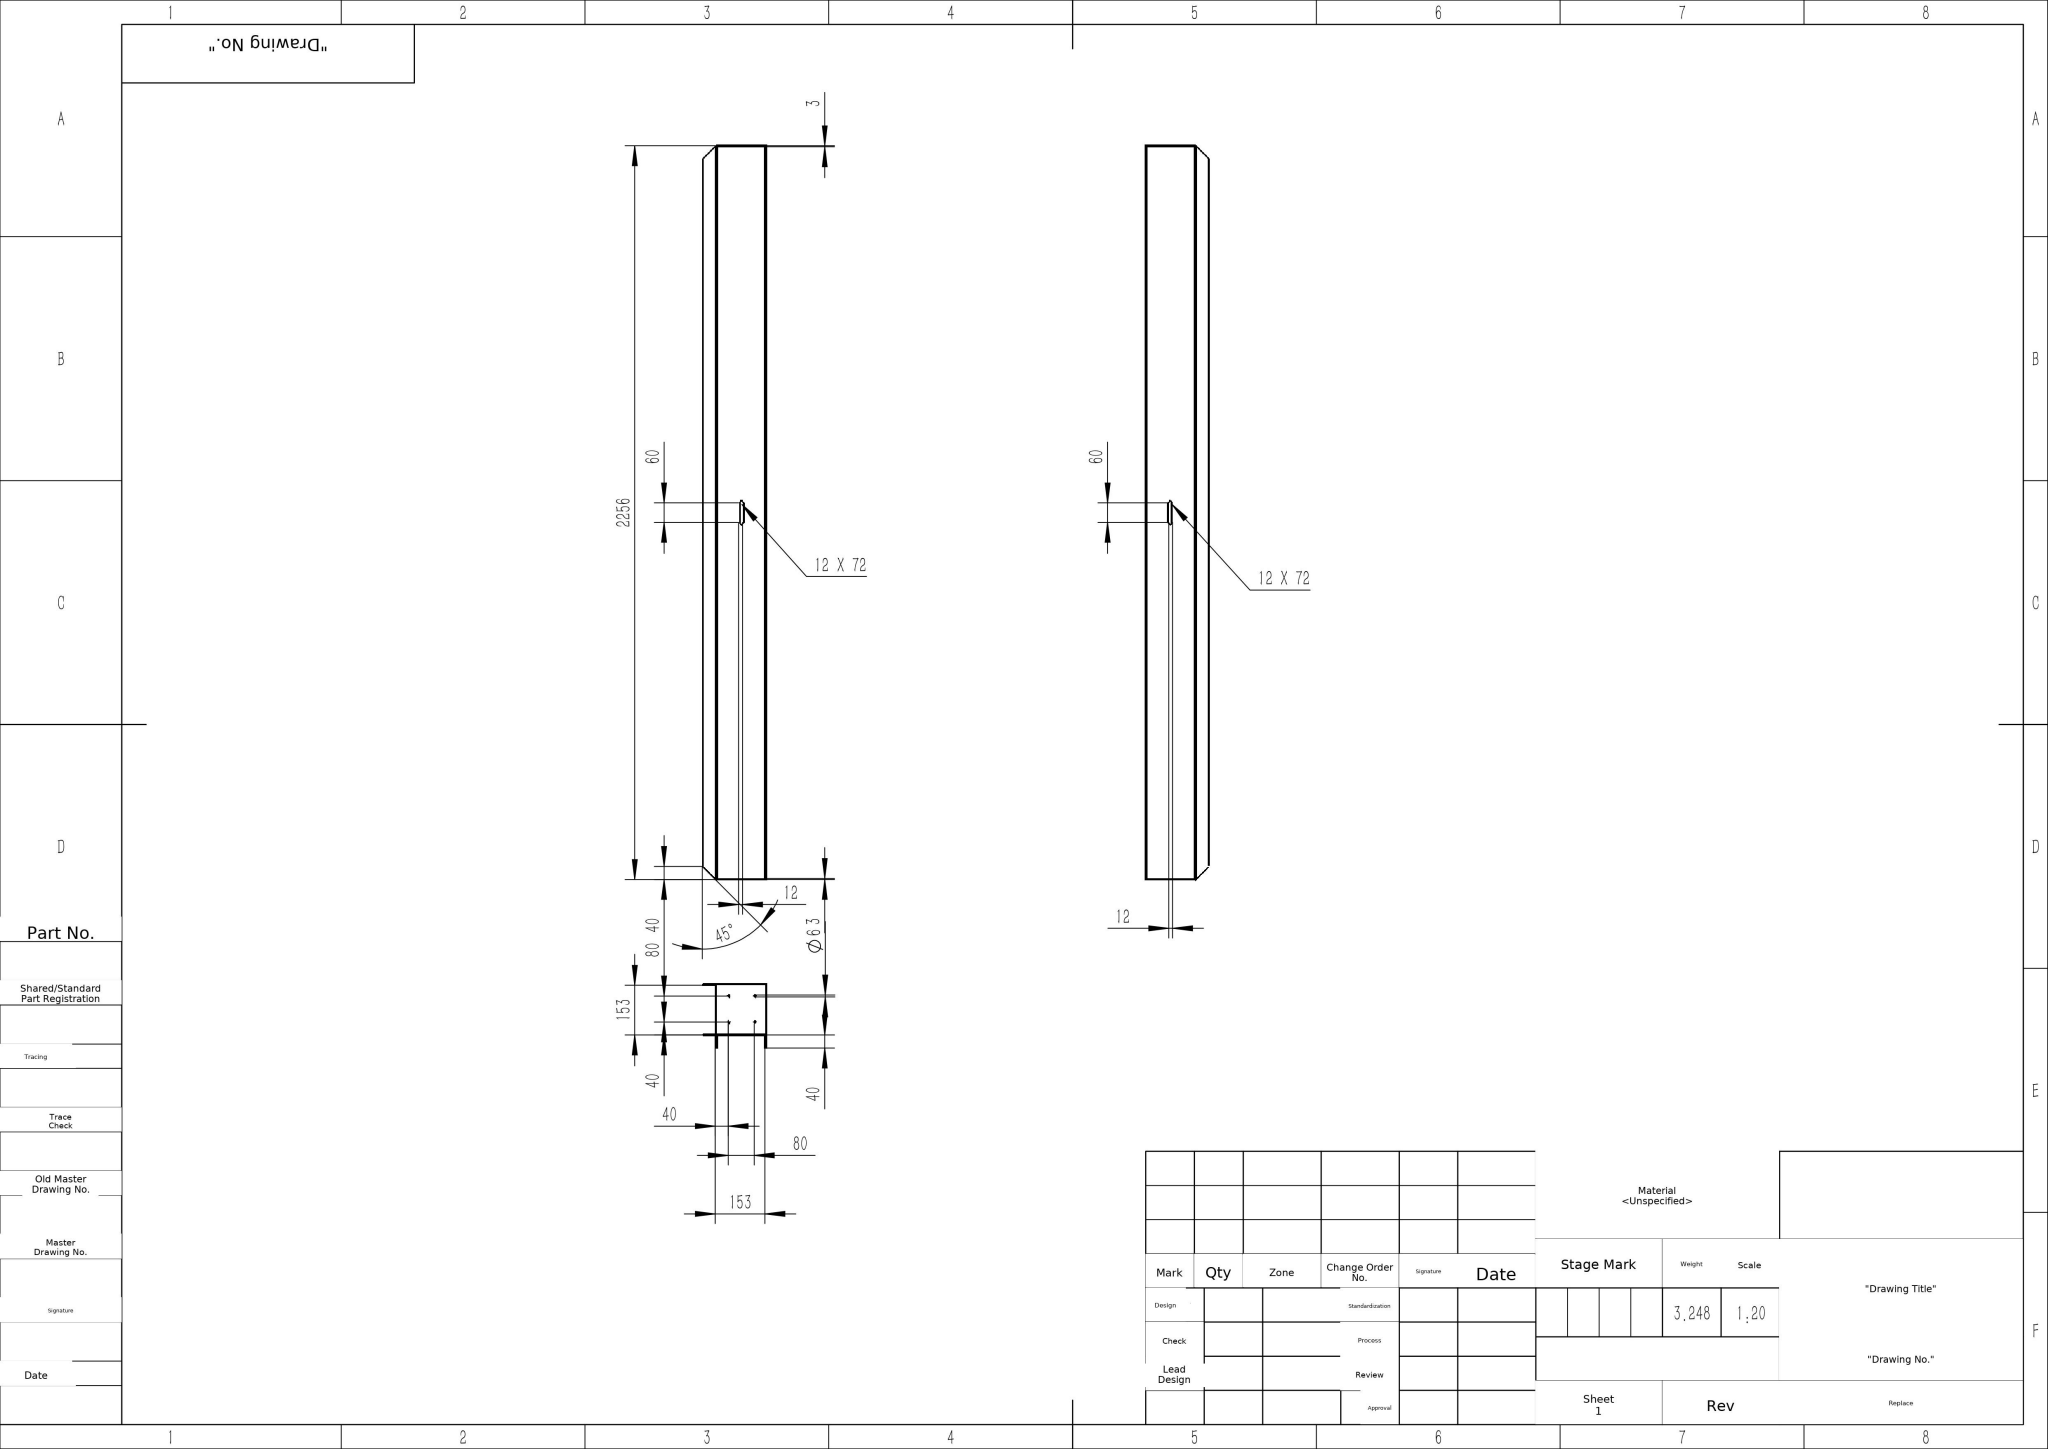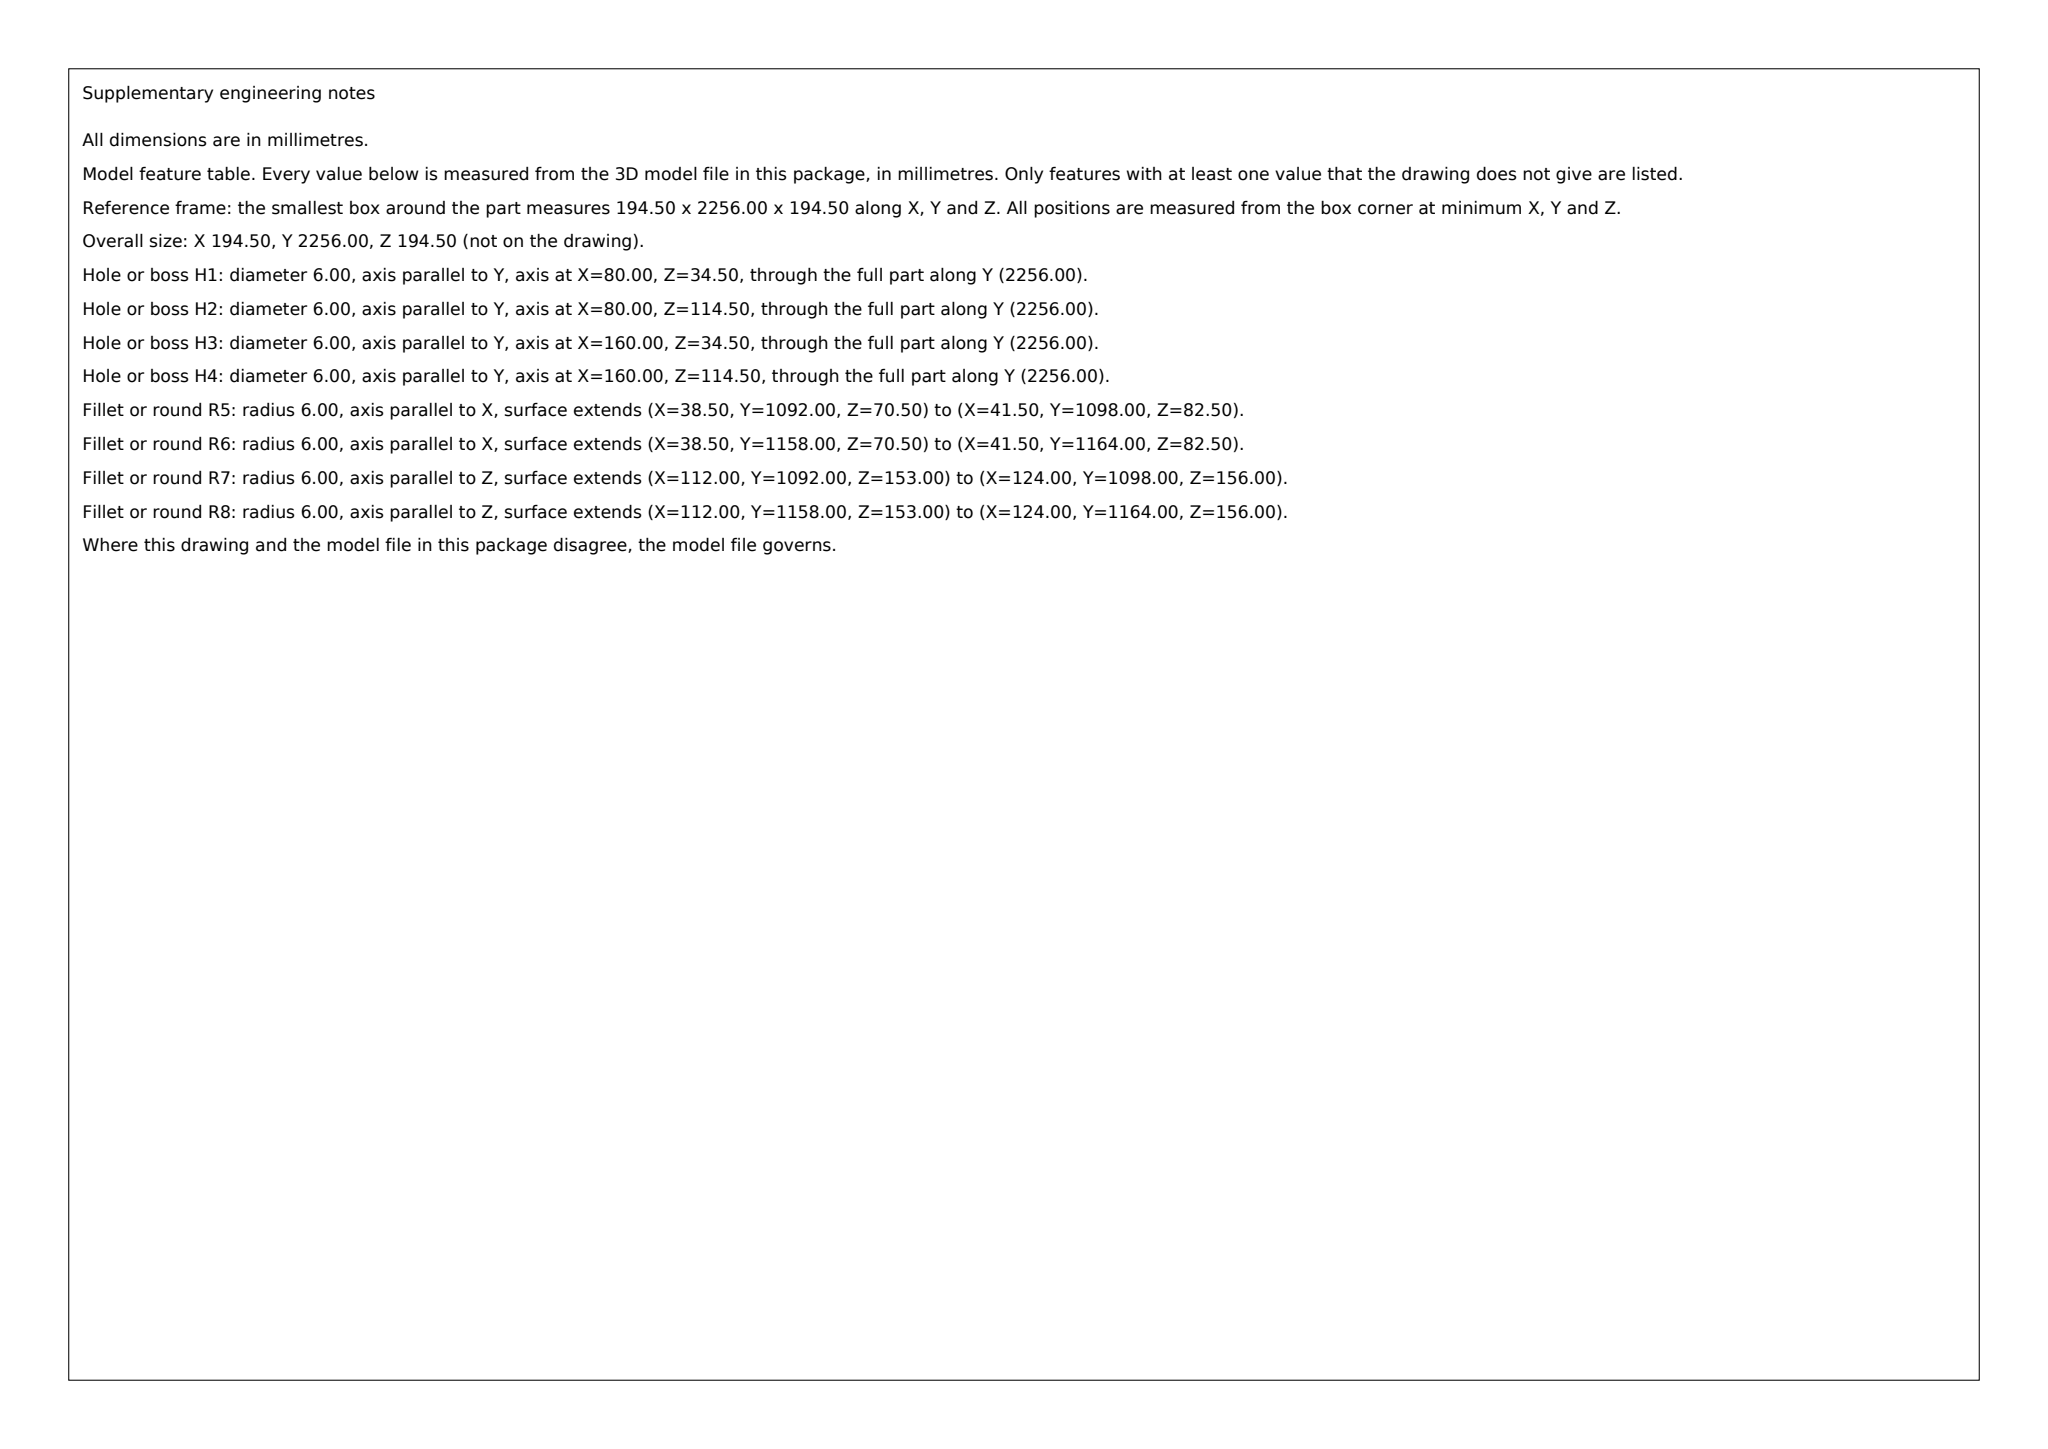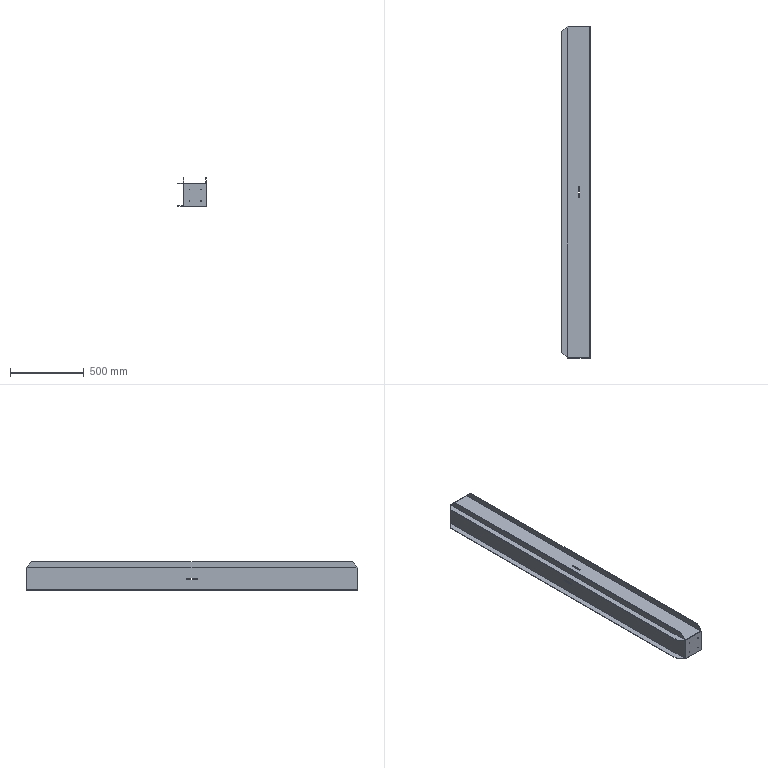Part | SolidWorks | mm | 1 solid | 48 faces | box 194.5 x 2256 x 194.5 mm | volume 3248488 mm3 | plane 28 | cylinder 20 | commonest cylinder face diameters 6 x16 12 x4